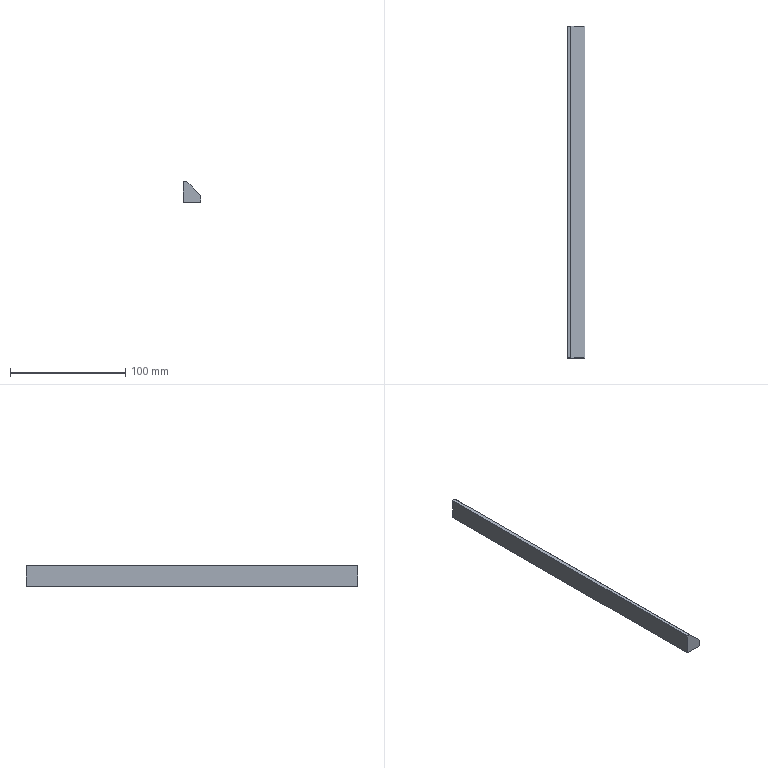Component | SolidWorks | 10-1111-1 | 1 solid | 19 faces | box 15 x 288 x 18 mm | volume 56756 mm3 | plane 7 | cylinder 6 | cone 6 | commonest cylinder face diameters 3.3 x6
build123d program:
from build123d import *

# Parameters (mm, degrees)
SKETCH1_2_W           = 15
SKETCH1_2_H           = 18
BOSS_EXTRUDE1_DEPTH   = 290
CHAMFER1_SIZE         = 12
LPATTERN2_COUNT       = 2
LPATTERN2_PITCH       = 120
LPATTERN2_COL_COUNT   = 2
LPATTERN2_COL_PITCH   = 120
SKETCH1_W             = 20
SKETCH1_H             = 24
TRIM_SEAT_ON_01_DEPTH = 2


with BuildPart() as part:
    # Sketch1_2 → Boss-Extrude1 (new body)
    with BuildSketch(Plane(origin=(0, 0, 0), x_dir=(1, 0, 0), z_dir=(0, 1, 0))):
        Rectangle(SKETCH1_2_W, SKETCH1_2_H)
    extrude(amount=BOSS_EXTRUDE1_DEPTH)

    # Chamfer1
    chamfer1_edges = [part.edges().sort_by_distance(p)[0] for p in [
        (-7.5, 145, 9),
    ]]
    chamfer(chamfer1_edges, length=CHAMFER1_SIZE)

    # Sketch5 → M4 Tapped Hole1 (revolve, cut)
    with BuildSketch(Plane(origin=(0, 145, -9), x_dir=(0, 1, 0), z_dir=(1, 0, 0))):
        Polygon((0, 0), (0, 11.091), (1.65, 10.1), (1.65, 0), align=None)
    m4_tapped_hole1 = revolve(axis=Axis((0, 145, -15.35), (0, 0, 1)), mode=Mode.SUBTRACT)

    # LPattern2: M4 Tapped Hole1 ×2
    with Locations(*[(0, i * LPATTERN2_PITCH, 0) for i in range(1, LPATTERN2_COUNT)]):
        add(m4_tapped_hole1, mode=Mode.SUBTRACT)

    # LPattern2 col: M4 Tapped Hole1 ×2
    with Locations(*[(0, -i * LPATTERN2_COL_PITCH, 0) for i in range(1, LPATTERN2_COL_COUNT)]):
        add(m4_tapped_hole1, mode=Mode.SUBTRACT)

    # Sketch1 → Trim-seat-on-01 (cut, symmetric)
    with BuildSketch(Plane(origin=(0, 290, 0), x_dir=(1, 0, 0), z_dir=(0, 1, 0))):
        Rectangle(SKETCH1_W, SKETCH1_H)
    extrude(amount=TRIM_SEAT_ON_01_DEPTH, both=True, mode=Mode.SUBTRACT)


solid = part.part

# Placed as in the assembly
solid = solid.moved(Location((-128.072, 696.224, 1291.056), (0, 0, 180)))
STEP:
#1=CARTESIAN_POINT('',(-5.107,16.977,50.872));
#2=VERTEX_POINT('',#1);
#3=CARTESIAN_POINT('',(-4.977,16.977,50.872));
#4=VERTEX_POINT('',#3);
#5=CARTESIAN_POINT('',(-5.042,16.977,50.872));
#6=DIRECTION('',(-0.,0.,-1.));
#7=DIRECTION('',(1.,0.,0.));
#8=AXIS2_PLACEMENT_3D('',#5,#6,#7);
#9=CIRCLE('',#8,0.06496);
#10=EDGE_CURVE('',#2,#4,#9,.T.);
#11=ORIENTED_EDGE('',*,*,#10,.F.);
#12=CARTESIAN_POINT('',(-5.107,16.977,50.475));
#13=VERTEX_POINT('',#12);
#14=CARTESIAN_POINT('',(-5.107,16.977,50.475));
#15=DIRECTION('',(-0.,0.,-1.));
#16=VECTOR('',#15,39.37);
#17=LINE('',#14,#16);
#18=EDGE_CURVE('',#2,#13,#17,.T.);
#19=ORIENTED_EDGE('',*,*,#18,.T.);
#20=CARTESIAN_POINT('',(-4.977,16.977,50.475));
#21=VERTEX_POINT('',#20);
#22=CARTESIAN_POINT('',(-5.042,16.977,50.475));
#23=DIRECTION('',(-0.,0.,-1.));
#24=DIRECTION('',(1.,0.,0.));
#25=AXIS2_PLACEMENT_3D('',#22,#23,#24);
#26=CIRCLE('',#25,0.06496);
#27=EDGE_CURVE('',#13,#21,#26,.T.);
#28=ORIENTED_EDGE('',*,*,#27,.T.);
#29=CARTESIAN_POINT('',(-4.977,16.977,50.475));
#30=DIRECTION('',(-0.,0.,-1.));
#31=VECTOR('',#30,39.37);
#32=LINE('',#29,#31);
#33=EDGE_CURVE('',#4,#21,#32,.T.);
#34=ORIENTED_EDGE('',*,*,#33,.F.);
#35=EDGE_LOOP('',(#11,#19,#28,#34));
#36=FACE_OUTER_BOUND('',#35,.T.);
#37=CARTESIAN_POINT('',(-5.042,16.977,50.475));
#38=DIRECTION('',(-0.,0.,-1.));
#39=DIRECTION('',(1.,0.,0.));
#40=AXIS2_PLACEMENT_3D('',#37,#38,#39);
#41=CYLINDRICAL_SURFACE('',#40,0.06496);
#42=ADVANCED_FACE('',(#36),#41,.F.);
#43=CARTESIAN_POINT('',(-5.042,16.977,50.911));
#44=VERTEX_POINT('',#43);
#45=CARTESIAN_POINT('',(-4.977,16.977,50.872));
#46=DIRECTION('',(0.8572,0.,-0.515));
#47=VECTOR('',#46,39.37);
#48=LINE('',#45,#47);
#49=EDGE_CURVE('',#44,#4,#48,.T.);
#50=ORIENTED_EDGE('',*,*,#49,.F.);
#51=CARTESIAN_POINT('',(-5.107,16.977,50.872));
#52=DIRECTION('',(-0.8572,0.,-0.515));
#53=VECTOR('',#52,39.37);
#54=LINE('',#51,#53);
#55=EDGE_CURVE('',#44,#2,#54,.T.);
#56=ORIENTED_EDGE('',*,*,#55,.T.);
#57=ORIENTED_EDGE('',*,*,#10,.T.);
#58=EDGE_LOOP('',(#50,#56,#57));
#59=FACE_OUTER_BOUND('',#58,.T.);
#60=CARTESIAN_POINT('',(-5.042,16.977,50.872));
#61=DIRECTION('',(-0.,0.,-1.));
#62=DIRECTION('',(1.,0.,0.));
#63=AXIS2_PLACEMENT_3D('',#60,#61,#62);
#64=CONICAL_SURFACE('',#63,0.06496,1.03);
#65=ADVANCED_FACE('',(#59),#64,.F.);
#66=CARTESIAN_POINT('',(-5.107,26.426,50.872));
#67=VERTEX_POINT('',#66);
#68=CARTESIAN_POINT('',(-4.977,26.426,50.872));
#69=VERTEX_POINT('',#68);
#70=CARTESIAN_POINT('',(-5.042,26.426,50.872));
#71=DIRECTION('',(-0.,0.,-1.));
#72=DIRECTION('',(1.,0.,0.));
#73=AXIS2_PLACEMENT_3D('',#70,#71,#72);
#74=CIRCLE('',#73,0.06496);
#75=EDGE_CURVE('',#67,#69,#74,.T.);
#76=ORIENTED_EDGE('',*,*,#75,.F.);
#77=CARTESIAN_POINT('',(-5.107,26.426,50.475));
#78=VERTEX_POINT('',#77);
#79=CARTESIAN_POINT('',(-5.107,26.426,50.475));
#80=DIRECTION('',(-0.,0.,-1.));
#81=VECTOR('',#80,39.37);
#82=LINE('',#79,#81);
#83=EDGE_CURVE('',#67,#78,#82,.T.);
#84=ORIENTED_EDGE('',*,*,#83,.T.);
#85=CARTESIAN_POINT('',(-4.977,26.426,50.475));
#86=VERTEX_POINT('',#85);
#87=CARTESIAN_POINT('',(-5.042,26.426,50.475));
#88=DIRECTION('',(-0.,0.,-1.));
#89=DIRECTION('',(1.,0.,0.));
#90=AXIS2_PLACEMENT_3D('',#87,#88,#89);
#91=CIRCLE('',#90,0.06496);
#92=EDGE_CURVE('',#78,#86,#91,.T.);
#93=ORIENTED_EDGE('',*,*,#92,.T.);
#94=CARTESIAN_POINT('',(-4.977,26.426,50.475));
#95=DIRECTION('',(-0.,0.,-1.));
#96=VECTOR('',#95,39.37);
#97=LINE('',#94,#96);
#98=EDGE_CURVE('',#69,#86,#97,.T.);
#99=ORIENTED_EDGE('',*,*,#98,.F.);
#100=EDGE_LOOP('',(#76,#84,#93,#99));
#101=FACE_OUTER_BOUND('',#100,.T.);
#102=CARTESIAN_POINT('',(-5.042,26.426,50.475));
#103=DIRECTION('',(-0.,0.,-1.));
#104=DIRECTION('',(1.,0.,0.));
#105=AXIS2_PLACEMENT_3D('',#102,#103,#104);
#106=CYLINDRICAL_SURFACE('',#105,0.06496);
#107=ADVANCED_FACE('',(#101),#106,.F.);
#108=CARTESIAN_POINT('',(-5.042,26.426,50.911));
#109=VERTEX_POINT('',#108);
#110=CARTESIAN_POINT('',(-4.977,26.426,50.872));
#111=DIRECTION('',(0.8572,0.,-0.515));
#112=VECTOR('',#111,39.37);
#113=LINE('',#110,#112);
#114=EDGE_CURVE('',#109,#69,#113,.T.);
#115=ORIENTED_EDGE('',*,*,#114,.F.);
#116=CARTESIAN_POINT('',(-5.107,26.426,50.872));
#117=DIRECTION('',(-0.8572,0.,-0.515));
#118=VECTOR('',#117,39.37);
#119=LINE('',#116,#118);
#120=EDGE_CURVE('',#109,#67,#119,.T.);
#121=ORIENTED_EDGE('',*,*,#120,.T.);
#122=ORIENTED_EDGE('',*,*,#75,.T.);
#123=EDGE_LOOP('',(#115,#121,#122));
#124=FACE_OUTER_BOUND('',#123,.T.);
#125=CARTESIAN_POINT('',(-5.042,26.426,50.872));
#126=DIRECTION('',(-0.,0.,-1.));
#127=DIRECTION('',(1.,0.,0.));
#128=AXIS2_PLACEMENT_3D('',#125,#126,#127);
#129=CONICAL_SURFACE('',#128,0.06496,1.03);
#130=ADVANCED_FACE('',(#124),#129,.F.);
#131=CARTESIAN_POINT('',(-5.107,21.702,50.872));
#132=VERTEX_POINT('',#131);
#133=CARTESIAN_POINT('',(-4.977,21.702,50.872));
#134=VERTEX_POINT('',#133);
#135=CARTESIAN_POINT('',(-5.042,21.702,50.872));
#136=DIRECTION('',(-0.,0.,-1.));
#137=DIRECTION('',(1.,0.,0.));
#138=AXIS2_PLACEMENT_3D('',#135,#136,#137);
#139=CIRCLE('',#138,0.06496);
#140=EDGE_CURVE('',#132,#134,#139,.T.);
#141=ORIENTED_EDGE('',*,*,#140,.F.);
#142=CARTESIAN_POINT('',(-5.107,21.702,50.475));
#143=VERTEX_POINT('',#142);
#144=CARTESIAN_POINT('',(-5.107,21.702,50.475));
#145=DIRECTION('',(-0.,0.,-1.));
#146=VECTOR('',#145,39.37);
#147=LINE('',#144,#146);
#148=EDGE_CURVE('',#132,#143,#147,.T.);
#149=ORIENTED_EDGE('',*,*,#148,.T.);
#150=CARTESIAN_POINT('',(-4.977,21.702,50.475));
#151=VERTEX_POINT('',#150);
#152=CARTESIAN_POINT('',(-5.042,21.702,50.475));
#153=DIRECTION('',(-0.,0.,-1.));
#154=DIRECTION('',(1.,0.,0.));
#155=AXIS2_PLACEMENT_3D('',#152,#153,#154);
#156=CIRCLE('',#155,0.06496);
#157=EDGE_CURVE('',#143,#151,#156,.T.);
#158=ORIENTED_EDGE('',*,*,#157,.T.);
#159=CARTESIAN_POINT('',(-4.977,21.702,50.475));
#160=DIRECTION('',(-0.,0.,-1.));
#161=VECTOR('',#160,39.37);
#162=LINE('',#159,#161);
#163=EDGE_CURVE('',#134,#151,#162,.T.);
#164=ORIENTED_EDGE('',*,*,#163,.F.);
#165=EDGE_LOOP('',(#141,#149,#158,#164));
#166=FACE_OUTER_BOUND('',#165,.T.);
#167=CARTESIAN_POINT('',(-5.042,21.702,50.475));
#168=DIRECTION('',(-0.,0.,-1.));
#169=DIRECTION('',(1.,0.,0.));
#170=AXIS2_PLACEMENT_3D('',#167,#168,#169);
#171=CYLINDRICAL_SURFACE('',#170,0.06496);
#172=ADVANCED_FACE('',(#166),#171,.F.);
#173=CARTESIAN_POINT('',(-5.042,21.702,50.911));
#174=VERTEX_POINT('',#173);
#175=CARTESIAN_POINT('',(-4.977,21.702,50.872));
#176=DIRECTION('',(0.8572,0.,-0.515));
#177=VECTOR('',#176,39.37);
#178=LINE('',#175,#177);
#179=EDGE_CURVE('',#174,#134,#178,.T.);
#180=ORIENTED_EDGE('',*,*,#179,.F.);
#181=CARTESIAN_POINT('',(-5.107,21.702,50.872));
#182=DIRECTION('',(-0.8572,0.,-0.515));
#183=VECTOR('',#182,39.37);
#184=LINE('',#181,#183);
#185=EDGE_CURVE('',#174,#132,#184,.T.);
#186=ORIENTED_EDGE('',*,*,#185,.T.);
#187=ORIENTED_EDGE('',*,*,#140,.T.);
#188=EDGE_LOOP('',(#180,#186,#187));
#189=FACE_OUTER_BOUND('',#188,.T.);
#190=CARTESIAN_POINT('',(-5.042,21.702,50.872));
#191=DIRECTION('',(-0.,0.,-1.));
#192=DIRECTION('',(1.,0.,0.));
#193=AXIS2_PLACEMENT_3D('',#190,#191,#192);
#194=CONICAL_SURFACE('',#193,0.06496,1.03);
#195=ADVANCED_FACE('',(#189),#194,.F.);
#196=CARTESIAN_POINT('',(-5.042,16.977,50.475));
#197=DIRECTION('',(-0.,0.,-1.));
#198=DIRECTION('',(1.,0.,0.));
#199=AXIS2_PLACEMENT_3D('',#196,#197,#198);
#200=CIRCLE('',#199,0.06496);
#201=EDGE_CURVE('',#21,#13,#200,.T.);
#202=ORIENTED_EDGE('',*,*,#201,.F.);
#203=ORIENTED_EDGE('',*,*,#27,.F.);
#204=EDGE_LOOP('',(#202,#203));
#205=FACE_BOUND('',#204,.T.);
#206=CARTESIAN_POINT('',(-5.042,26.426,50.475));
#207=DIRECTION('',(-0.,0.,-1.));
#208=DIRECTION('',(1.,0.,0.));
#209=AXIS2_PLACEMENT_3D('',#206,#207,#208);
#210=CIRCLE('',#209,0.06496);
#211=EDGE_CURVE('',#86,#78,#210,.T.);
#212=ORIENTED_EDGE('',*,*,#211,.F.);
#213=ORIENTED_EDGE('',*,*,#92,.F.);
#214=EDGE_LOOP('',(#212,#213));
#215=FACE_BOUND('',#214,.T.);
#216=CARTESIAN_POINT('',(-4.747,16.072,50.475));
#217=VERTEX_POINT('',#216);
#218=CARTESIAN_POINT('',(-4.747,27.41,50.475));
#219=VERTEX_POINT('',#218);
#220=CARTESIAN_POINT('',(-4.747,15.993,50.475));
#221=DIRECTION('',(-0.,1.,0.));
#222=VECTOR('',#221,39.37);
#223=LINE('',#220,#222);
#224=EDGE_CURVE('',#217,#219,#223,.T.);
#225=ORIENTED_EDGE('',*,*,#224,.F.);
#226=CARTESIAN_POINT('',(-5.337,16.072,50.475));
#227=VERTEX_POINT('',#226);
#228=CARTESIAN_POINT('',(-5.337,16.072,50.475));
#229=DIRECTION('',(-1.,-0.,0.));
#230=VECTOR('',#229,39.37);
#231=LINE('',#228,#230);
#232=EDGE_CURVE('',#217,#227,#231,.T.);
#233=ORIENTED_EDGE('',*,*,#232,.T.);
#234=CARTESIAN_POINT('',(-5.337,27.41,50.475));
#235=VERTEX_POINT('',#234);
#236=CARTESIAN_POINT('',(-5.337,15.993,50.475));
#237=DIRECTION('',(-0.,1.,0.));
#238=VECTOR('',#237,39.37);
#239=LINE('',#236,#238);
#240=EDGE_CURVE('',#227,#235,#239,.T.);
#241=ORIENTED_EDGE('',*,*,#240,.T.);
#242=CARTESIAN_POINT('',(-5.337,27.41,50.475));
#243=DIRECTION('',(1.,0.,-0.));
#244=VECTOR('',#243,39.37);
#245=LINE('',#242,#244);
#246=EDGE_CURVE('',#235,#219,#245,.T.);
#247=ORIENTED_EDGE('',*,*,#246,.T.);
#248=EDGE_LOOP('',(#225,#233,#241,#247));
#249=FACE_OUTER_BOUND('',#248,.T.);
#250=CARTESIAN_POINT('',(-5.042,21.702,50.475));
#251=DIRECTION('',(-0.,0.,-1.));
#252=DIRECTION('',(1.,0.,0.));
#253=AXIS2_PLACEMENT_3D('',#250,#251,#252);
#254=CIRCLE('',#253,0.06496);
#255=EDGE_CURVE('',#151,#143,#254,.T.);
#256=ORIENTED_EDGE('',*,*,#255,.F.);
#257=ORIENTED_EDGE('',*,*,#157,.F.);
#258=EDGE_LOOP('',(#256,#257));
#259=FACE_BOUND('',#258,.T.);
#260=CARTESIAN_POINT('',(-5.337,15.993,50.475));
#261=DIRECTION('',(0.,-0.,1.));
#262=DIRECTION('',(-1.,-0.,0.));
#263=AXIS2_PLACEMENT_3D('',#260,#261,#262);
#264=PLANE('',#263);
#265=ADVANCED_FACE('',(#205,#215,#249,#259),#264,.F.);
#266=CARTESIAN_POINT('',(-4.747,27.41,50.711));
#267=VERTEX_POINT('',#266);
#268=CARTESIAN_POINT('',(-4.747,16.072,50.711));
#269=VERTEX_POINT('',#268);
#270=CARTESIAN_POINT('',(-4.747,15.993,50.711));
#271=DIRECTION('',(0.,-1.,-0.));
#272=VECTOR('',#271,39.37);
#273=LINE('',#270,#272);
#274=EDGE_CURVE('',#267,#269,#273,.T.);
#275=ORIENTED_EDGE('',*,*,#274,.T.);
#276=CARTESIAN_POINT('',(-4.747,16.072,50.475));
#277=DIRECTION('',(0.,0.,-1.));
#278=VECTOR('',#277,39.37);
#279=LINE('',#276,#278);
#280=EDGE_CURVE('',#269,#217,#279,.T.);
#281=ORIENTED_EDGE('',*,*,#280,.T.);
#282=ORIENTED_EDGE('',*,*,#224,.T.);
#283=CARTESIAN_POINT('',(-4.747,27.41,50.475));
#284=DIRECTION('',(-0.,-0.,1.));
#285=VECTOR('',#284,39.37);
#286=LINE('',#283,#285);
#287=EDGE_CURVE('',#219,#267,#286,.T.);
#288=ORIENTED_EDGE('',*,*,#287,.T.);
#289=EDGE_LOOP('',(#275,#281,#282,#288));
#290=FACE_OUTER_BOUND('',#289,.T.);
#291=CARTESIAN_POINT('',(-4.747,15.993,50.475));
#292=DIRECTION('',(-1.,-0.,-0.));
#293=DIRECTION('',(0.,0.,-1.));
#294=AXIS2_PLACEMENT_3D('',#291,#292,#293);
#295=PLANE('',#294);
#296=ADVANCED_FACE('',(#290),#295,.F.);
#297=CARTESIAN_POINT('',(-5.337,16.072,51.183));
#298=VERTEX_POINT('',#297);
#299=CARTESIAN_POINT('',(-5.337,27.41,51.183));
#300=VERTEX_POINT('',#299);
#301=CARTESIAN_POINT('',(-5.337,15.993,51.183));
#302=DIRECTION('',(-0.,1.,0.));
#303=VECTOR('',#302,39.37);
#304=LINE('',#301,#303);
#305=EDGE_CURVE('',#298,#300,#304,.T.);
#306=ORIENTED_EDGE('',*,*,#305,.F.);
#307=CARTESIAN_POINT('',(-5.219,16.072,51.183));
#308=VERTEX_POINT('',#307);
#309=CARTESIAN_POINT('',(-5.337,16.072,51.183));
#310=DIRECTION('',(1.,0.,-0.));
#311=VECTOR('',#310,39.37);
#312=LINE('',#309,#311);
#313=EDGE_CURVE('',#298,#308,#312,.T.);
#314=ORIENTED_EDGE('',*,*,#313,.T.);
#315=CARTESIAN_POINT('',(-5.219,27.41,51.183));
#316=VERTEX_POINT('',#315);
#317=CARTESIAN_POINT('',(-5.219,15.993,51.183));
#318=DIRECTION('',(-0.,1.,0.));
#319=VECTOR('',#318,39.37);
#320=LINE('',#317,#319);
#321=EDGE_CURVE('',#308,#316,#320,.T.);
#322=ORIENTED_EDGE('',*,*,#321,.T.);
#323=CARTESIAN_POINT('',(-5.337,27.41,51.183));
#324=DIRECTION('',(-1.,-0.,0.));
#325=VECTOR('',#324,39.37);
#326=LINE('',#323,#325);
#327=EDGE_CURVE('',#316,#300,#326,.T.);
#328=ORIENTED_EDGE('',*,*,#327,.T.);
#329=EDGE_LOOP('',(#306,#314,#322,#328));
#330=FACE_OUTER_BOUND('',#329,.T.);
#331=CARTESIAN_POINT('',(-5.337,15.993,51.183));
#332=DIRECTION('',(-0.,0.,-1.));
#333=DIRECTION('',(1.,0.,-0.));
#334=AXIS2_PLACEMENT_3D('',#331,#332,#333);
#335=PLANE('',#334);
#336=ADVANCED_FACE('',(#330),#335,.F.);
#337=ORIENTED_EDGE('',*,*,#240,.F.);
#338=CARTESIAN_POINT('',(-5.337,16.072,50.475));
#339=DIRECTION('',(0.,-0.,1.));
#340=VECTOR('',#339,39.37);
#341=LINE('',#338,#340);
#342=EDGE_CURVE('',#227,#298,#341,.T.);
#343=ORIENTED_EDGE('',*,*,#342,.T.);
#344=ORIENTED_EDGE('',*,*,#305,.T.);
#345=CARTESIAN_POINT('',(-5.337,27.41,50.475));
#346=DIRECTION('',(-0.,0.,-1.));
#347=VECTOR('',#346,39.37);
#348=LINE('',#345,#347);
#349=EDGE_CURVE('',#300,#235,#348,.T.);
#350=ORIENTED_EDGE('',*,*,#349,.T.);
#351=EDGE_LOOP('',(#337,#343,#344,#350));
#352=FACE_OUTER_BOUND('',#351,.T.);
#353=CARTESIAN_POINT('',(-5.337,15.993,50.475));
#354=DIRECTION('',(1.,0.,-0.));
#355=DIRECTION('',(0.,-0.,1.));
#356=AXIS2_PLACEMENT_3D('',#353,#354,#355);
#357=PLANE('',#356);
#358=ADVANCED_FACE('',(#352),#357,.F.);
#359=ORIENTED_EDGE('',*,*,#327,.F.);
#360=CARTESIAN_POINT('',(-4.954,27.41,50.918));
#361=DIRECTION('',(0.7071,0.,-0.7071));
#362=VECTOR('',#361,39.37);
#363=LINE('',#360,#362);
#364=EDGE_CURVE('',#316,#267,#363,.T.);
#365=ORIENTED_EDGE('',*,*,#364,.T.);
#366=ORIENTED_EDGE('',*,*,#287,.F.);
#367=ORIENTED_EDGE('',*,*,#246,.F.);
#368=ORIENTED_EDGE('',*,*,#349,.F.);
#369=EDGE_LOOP('',(#359,#365,#366,#367,#368));
#370=FACE_OUTER_BOUND('',#369,.T.);
#371=CARTESIAN_POINT('',(-5.042,27.41,50.829));
#372=DIRECTION('',(-0.,1.,0.));
#373=DIRECTION('',(-0.,0.,-1.));
#374=AXIS2_PLACEMENT_3D('',#371,#372,#373);
#375=PLANE('',#374);
#376=ADVANCED_FACE('',(#370),#375,.T.);
#377=CARTESIAN_POINT('',(-5.219,16.072,51.183));
#378=DIRECTION('',(-0.7071,-0.,0.7071));
#379=VECTOR('',#378,39.37);
#380=LINE('',#377,#379);
#381=EDGE_CURVE('',#269,#308,#380,.T.);
#382=ORIENTED_EDGE('',*,*,#381,.F.);
#383=ORIENTED_EDGE('',*,*,#274,.F.);
#384=ORIENTED_EDGE('',*,*,#364,.F.);
#385=ORIENTED_EDGE('',*,*,#321,.F.);
#386=EDGE_LOOP('',(#382,#383,#384,#385));
#387=FACE_OUTER_BOUND('',#386,.T.);
#388=CARTESIAN_POINT('',(-5.219,15.993,51.183));
#389=DIRECTION('',(-0.7071,0.,-0.7071));
#390=DIRECTION('',(-0.,1.,0.));
#391=AXIS2_PLACEMENT_3D('',#388,#389,#390);
#392=PLANE('',#391);
#393=ADVANCED_FACE('',(#387),#392,.F.);
#394=ORIENTED_EDGE('',*,*,#185,.F.);
#395=ORIENTED_EDGE('',*,*,#179,.T.);
#396=CARTESIAN_POINT('',(-5.042,21.702,50.872));
#397=DIRECTION('',(-0.,0.,-1.));
#398=DIRECTION('',(1.,0.,0.));
#399=AXIS2_PLACEMENT_3D('',#396,#397,#398);
#400=CIRCLE('',#399,0.06496);
#401=EDGE_CURVE('',#134,#132,#400,.T.);
#402=ORIENTED_EDGE('',*,*,#401,.T.);
#403=EDGE_LOOP('',(#394,#395,#402));
#404=FACE_OUTER_BOUND('',#403,.T.);
#405=CARTESIAN_POINT('',(-5.042,21.702,50.872));
#406=DIRECTION('',(-0.,0.,-1.));
#407=DIRECTION('',(1.,0.,0.));
#408=AXIS2_PLACEMENT_3D('',#405,#406,#407);
#409=CONICAL_SURFACE('',#408,0.06496,1.03);
#410=ADVANCED_FACE('',(#404),#409,.F.);
#411=ORIENTED_EDGE('',*,*,#148,.F.);
#412=ORIENTED_EDGE('',*,*,#401,.F.);
#413=ORIENTED_EDGE('',*,*,#163,.T.);
#414=ORIENTED_EDGE('',*,*,#255,.T.);
#415=EDGE_LOOP('',(#411,#412,#413,#414));
#416=FACE_OUTER_BOUND('',#415,.T.);
#417=CARTESIAN_POINT('',(-5.042,21.702,50.475));
#418=DIRECTION('',(-0.,0.,-1.));
#419=DIRECTION('',(1.,0.,0.));
#420=AXIS2_PLACEMENT_3D('',#417,#418,#419);
#421=CYLINDRICAL_SURFACE('',#420,0.06496);
#422=ADVANCED_FACE('',(#416),#421,.F.);
#423=ORIENTED_EDGE('',*,*,#120,.F.);
#424=ORIENTED_EDGE('',*,*,#114,.T.);
#425=CARTESIAN_POINT('',(-5.042,26.426,50.872));
#426=DIRECTION('',(-0.,0.,-1.));
#427=DIRECTION('',(1.,0.,0.));
#428=AXIS2_PLACEMENT_3D('',#425,#426,#427);
#429=CIRCLE('',#428,0.06496);
#430=EDGE_CURVE('',#69,#67,#429,.T.);
#431=ORIENTED_EDGE('',*,*,#430,.T.);
#432=EDGE_LOOP('',(#423,#424,#431));
#433=FACE_OUTER_BOUND('',#432,.T.);
#434=CARTESIAN_POINT('',(-5.042,26.426,50.872));
#435=DIRECTION('',(-0.,0.,-1.));
#436=DIRECTION('',(1.,0.,0.));
#437=AXIS2_PLACEMENT_3D('',#434,#435,#436);
#438=CONICAL_SURFACE('',#437,0.06496,1.03);
#439=ADVANCED_FACE('',(#433),#438,.F.);
#440=ORIENTED_EDGE('',*,*,#83,.F.);
#441=ORIENTED_EDGE('',*,*,#430,.F.);
#442=ORIENTED_EDGE('',*,*,#98,.T.);
#443=ORIENTED_EDGE('',*,*,#211,.T.);
#444=EDGE_LOOP('',(#440,#441,#442,#443));
#445=FACE_OUTER_BOUND('',#444,.T.);
#446=CARTESIAN_POINT('',(-5.042,26.426,50.475));
#447=DIRECTION('',(-0.,0.,-1.));
#448=DIRECTION('',(1.,0.,0.));
#449=AXIS2_PLACEMENT_3D('',#446,#447,#448);
#450=CYLINDRICAL_SURFACE('',#449,0.06496);
#451=ADVANCED_FACE('',(#445),#450,.F.);
#452=ORIENTED_EDGE('',*,*,#55,.F.);
#453=ORIENTED_EDGE('',*,*,#49,.T.);
#454=CARTESIAN_POINT('',(-5.042,16.977,50.872));
#455=DIRECTION('',(-0.,0.,-1.));
#456=DIRECTION('',(1.,0.,0.));
#457=AXIS2_PLACEMENT_3D('',#454,#455,#456);
#458=CIRCLE('',#457,0.06496);
#459=EDGE_CURVE('',#4,#2,#458,.T.);
#460=ORIENTED_EDGE('',*,*,#459,.T.);
#461=EDGE_LOOP('',(#452,#453,#460));
#462=FACE_OUTER_BOUND('',#461,.T.);
#463=CARTESIAN_POINT('',(-5.042,16.977,50.872));
#464=DIRECTION('',(-0.,0.,-1.));
#465=DIRECTION('',(1.,0.,0.));
#466=AXIS2_PLACEMENT_3D('',#463,#464,#465);
#467=CONICAL_SURFACE('',#466,0.06496,1.03);
#468=ADVANCED_FACE('',(#462),#467,.F.);
#469=ORIENTED_EDGE('',*,*,#18,.F.);
#470=ORIENTED_EDGE('',*,*,#459,.F.);
#471=ORIENTED_EDGE('',*,*,#33,.T.);
#472=ORIENTED_EDGE('',*,*,#201,.T.);
#473=EDGE_LOOP('',(#469,#470,#471,#472));
#474=FACE_OUTER_BOUND('',#473,.T.);
#475=CARTESIAN_POINT('',(-5.042,16.977,50.475));
#476=DIRECTION('',(-0.,0.,-1.));
#477=DIRECTION('',(1.,0.,0.));
#478=AXIS2_PLACEMENT_3D('',#475,#476,#477);
#479=CYLINDRICAL_SURFACE('',#478,0.06496);
#480=ADVANCED_FACE('',(#474),#479,.F.);
#481=ORIENTED_EDGE('',*,*,#232,.F.);
#482=ORIENTED_EDGE('',*,*,#280,.F.);
#483=ORIENTED_EDGE('',*,*,#381,.T.);
#484=ORIENTED_EDGE('',*,*,#313,.F.);
#485=ORIENTED_EDGE('',*,*,#342,.F.);
#486=EDGE_LOOP('',(#481,#482,#483,#484,#485));
#487=FACE_OUTER_BOUND('',#486,.T.);
#488=CARTESIAN_POINT('',(-5.042,16.072,50.829));
#489=DIRECTION('',(-0.,1.,0.));
#490=DIRECTION('',(-0.,0.,-1.));
#491=AXIS2_PLACEMENT_3D('',#488,#489,#490);
#492=PLANE('',#491);
#493=ADVANCED_FACE('',(#487),#492,.F.);
#494=CLOSED_SHELL('',(#42,#65,#107,#130,#172,#195,#265,#296,#336,#358,#376,#393,#410,#422,#439,#451,#468,#480,#493));
#495=MANIFOLD_SOLID_BREP('',#494);
#496=CARTESIAN_POINT('',(0.,0.,0.));
#497=DIRECTION('',(0.,0.,1.));
#498=DIRECTION('',(1.,0.,0.));
#499=AXIS2_PLACEMENT_3D('',#496,#497,#498);
#500=(LENGTH_UNIT()NAMED_UNIT(*)SI_UNIT($,.METRE.));
#501=LENGTH_MEASURE_WITH_UNIT(LENGTH_MEASURE(0.0254),#500);
#502=DIMENSIONAL_EXPONENTS(1.,0.,0.,0.,0.,0.,0.);
#503=(CONVERSION_BASED_UNIT('',#501)LENGTH_UNIT()NAMED_UNIT(#502));
#504=UNCERTAINTY_MEASURE_WITH_UNIT(LENGTH_MEASURE(0.00001),#503,'','');
#505=(NAMED_UNIT(*)PLANE_ANGLE_UNIT()SI_UNIT($,.RADIAN.));
#506=(NAMED_UNIT(*)SI_UNIT($,.STERADIAN.)SOLID_ANGLE_UNIT());
#507=(GEOMETRIC_REPRESENTATION_CONTEXT(3)GLOBAL_UNCERTAINTY_ASSIGNED_CONTEXT((#504))GLOBAL_UNIT_ASSIGNED_CONTEXT((#503,#505,#506))REPRESENTATION_CONTEXT('',''));
#508=ADVANCED_BREP_SHAPE_REPRESENTATION('',(#495,#499),#507);
#509=COLOUR_RGB('',0.7922,0.8196,0.9333);
#510=FILL_AREA_STYLE_COLOUR('',#509);
#511=FILL_AREA_STYLE('',(#510));
#512=SURFACE_STYLE_FILL_AREA(#511);
#513=SURFACE_SIDE_STYLE('',(#512));
#514=SURFACE_STYLE_USAGE(.BOTH.,#513);
#515=PRESENTATION_STYLE_ASSIGNMENT((#514));
#516=STYLED_ITEM('',(#515),#495);
#517=PRESENTATION_LAYER_ASSIGNMENT('','',(#516));
#518=(LENGTH_UNIT()NAMED_UNIT(*)SI_UNIT($,.METRE.));
#519=LENGTH_MEASURE_WITH_UNIT(LENGTH_MEASURE(0.0254),#518);
#520=DIMENSIONAL_EXPONENTS(1.,0.,0.,0.,0.,0.,0.);
#521=(CONVERSION_BASED_UNIT('',#519)LENGTH_UNIT()NAMED_UNIT(#520));
#522=UNCERTAINTY_MEASURE_WITH_UNIT(LENGTH_MEASURE(0.00001),#521,'','');
#523=(NAMED_UNIT(*)PLANE_ANGLE_UNIT()SI_UNIT($,.RADIAN.));
#524=(NAMED_UNIT(*)SI_UNIT($,.STERADIAN.)SOLID_ANGLE_UNIT());
#525=(GEOMETRIC_REPRESENTATION_CONTEXT(3)GLOBAL_UNCERTAINTY_ASSIGNED_CONTEXT((#522))GLOBAL_UNIT_ASSIGNED_CONTEXT((#521,#523,#524))REPRESENTATION_CONTEXT('',''));
#526=MECHANICAL_DESIGN_GEOMETRIC_PRESENTATION_REPRESENTATION('',(#516),#525);